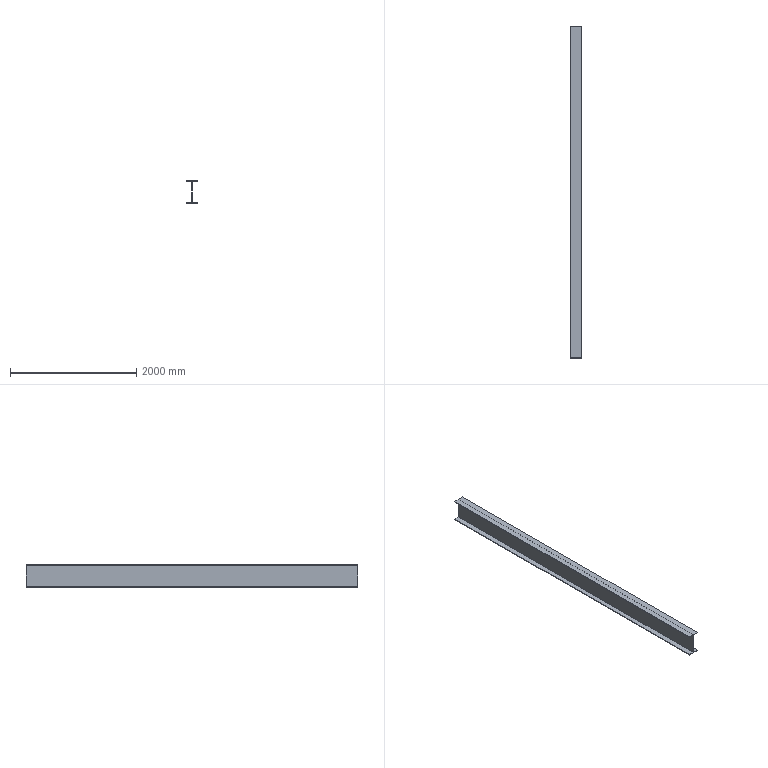Component | NX | ZHIJIA11 | 1 solid | 14 faces | box 175 x 5250 x 350 mm | volume 35700000 mm3 | plane 14
STEP:
#1=CARTESIAN_POINT('',(0.,0.,0.));
#2=DIRECTION('',(0.,0.,1.));
#3=DIRECTION('',(1.,0.,0.));
#4=AXIS2_PLACEMENT_3D('',#1,#2,#3);
#5=CARTESIAN_POINT('',(2412.5,2625.,3538.094));
#6=VERTEX_POINT('',#5);
#7=CARTESIAN_POINT('',(2412.5,2625.,3528.094));
#8=VERTEX_POINT('',#7);
#9=CARTESIAN_POINT('',(2412.5,2625.,3538.094));
#10=DIRECTION('',(-0.,0.,-1.));
#11=VECTOR('',#10,1.);
#12=LINE('',#9,#11);
#13=CARTESIAN_POINT('',(2412.5,-2625.,3538.094));
#14=DIRECTION('',(1.,0.,-0.));
#15=DIRECTION('',(0.,0.,1.));
#16=AXIS2_PLACEMENT_3D('',#13,#14,#15);
#17=PLANE('',#16);
#18=CARTESIAN_POINT('',(0.,-5250.));
#19=DIRECTION('',(-1.,0.));
#20=VECTOR('',#19,1.);
#21=LINE('',#18,#20);
#22=(GEOMETRIC_REPRESENTATION_CONTEXT(2)PARAMETRIC_REPRESENTATION_CONTEXT()REPRESENTATION_CONTEXT('',''));
#23=DEFINITIONAL_REPRESENTATION('',(#21),#22);
#24=PCURVE('',#17,#23);
#25=CARTESIAN_POINT('',(2412.5,2625.,3528.094));
#26=DIRECTION('',(0.,-1.,0.));
#27=DIRECTION('',(1.,0.,0.));
#28=AXIS2_PLACEMENT_3D('',#25,#26,#27);
#29=PLANE('',#28);
#30=CARTESIAN_POINT('',(0.,10.));
#31=DIRECTION('',(-0.,-1.));
#32=VECTOR('',#31,1.);
#33=LINE('',#30,#32);
#34=(GEOMETRIC_REPRESENTATION_CONTEXT(2)PARAMETRIC_REPRESENTATION_CONTEXT()REPRESENTATION_CONTEXT('',''));
#35=DEFINITIONAL_REPRESENTATION('',(#33),#34);
#36=PCURVE('',#29,#35);
#37=SURFACE_CURVE('',#12,(#24,#36),.PCURVE_S1.);
#38=EDGE_CURVE('',#6,#8,#37,.T.);
#39=ORIENTED_EDGE('',*,*,#38,.T.);
#40=CARTESIAN_POINT('',(2412.5,-2625.,3528.094));
#41=VERTEX_POINT('',#40);
#42=CARTESIAN_POINT('',(2412.5,-2625.,3528.094));
#43=DIRECTION('',(0.,1.,0.));
#44=VECTOR('',#43,1.);
#45=LINE('',#42,#44);
#46=CARTESIAN_POINT('',(-10.,0.));
#47=DIRECTION('',(0.,-1.));
#48=VECTOR('',#47,1.);
#49=LINE('',#46,#48);
#50=(GEOMETRIC_REPRESENTATION_CONTEXT(2)PARAMETRIC_REPRESENTATION_CONTEXT()REPRESENTATION_CONTEXT('',''));
#51=DEFINITIONAL_REPRESENTATION('',(#49),#50);
#52=PCURVE('',#17,#51);
#53=CARTESIAN_POINT('',(2412.5,-2625.,3528.094));
#54=DIRECTION('',(0.,0.,1.));
#55=DIRECTION('',(0.,-1.,0.));
#56=AXIS2_PLACEMENT_3D('',#53,#54,#55);
#57=PLANE('',#56);
#58=CARTESIAN_POINT('',(0.,0.));
#59=DIRECTION('',(-1.,0.));
#60=VECTOR('',#59,1.);
#61=LINE('',#58,#60);
#62=(GEOMETRIC_REPRESENTATION_CONTEXT(2)PARAMETRIC_REPRESENTATION_CONTEXT()REPRESENTATION_CONTEXT('',''));
#63=DEFINITIONAL_REPRESENTATION('',(#61),#62);
#64=PCURVE('',#57,#63);
#65=SURFACE_CURVE('',#45,(#52,#64),.PCURVE_S1.);
#66=EDGE_CURVE('',#41,#8,#65,.T.);
#67=ORIENTED_EDGE('',*,*,#66,.F.);
#68=CARTESIAN_POINT('',(2412.5,-2625.,3538.094));
#69=VERTEX_POINT('',#68);
#70=CARTESIAN_POINT('',(2412.5,-2625.,3538.094));
#71=DIRECTION('',(-0.,0.,-1.));
#72=VECTOR('',#71,1.);
#73=LINE('',#70,#72);
#74=CARTESIAN_POINT('',(0.,0.));
#75=DIRECTION('',(-1.,0.));
#76=VECTOR('',#75,1.);
#77=LINE('',#74,#76);
#78=(GEOMETRIC_REPRESENTATION_CONTEXT(2)PARAMETRIC_REPRESENTATION_CONTEXT()REPRESENTATION_CONTEXT('',''));
#79=DEFINITIONAL_REPRESENTATION('',(#77),#78);
#80=PCURVE('',#17,#79);
#81=CARTESIAN_POINT('',(2412.5,-2625.,3528.094));
#82=DIRECTION('',(0.,-1.,0.));
#83=DIRECTION('',(1.,0.,0.));
#84=AXIS2_PLACEMENT_3D('',#81,#82,#83);
#85=PLANE('',#84);
#86=CARTESIAN_POINT('',(0.,10.));
#87=DIRECTION('',(-0.,-1.));
#88=VECTOR('',#87,1.);
#89=LINE('',#86,#88);
#90=(GEOMETRIC_REPRESENTATION_CONTEXT(2)PARAMETRIC_REPRESENTATION_CONTEXT()REPRESENTATION_CONTEXT('',''));
#91=DEFINITIONAL_REPRESENTATION('',(#89),#90);
#92=PCURVE('',#85,#91);
#93=SURFACE_CURVE('',#73,(#80,#92),.PCURVE_S1.);
#94=EDGE_CURVE('',#69,#41,#93,.T.);
#95=ORIENTED_EDGE('',*,*,#94,.F.);
#96=CARTESIAN_POINT('',(2412.5,-2625.,3538.094));
#97=DIRECTION('',(0.,1.,0.));
#98=VECTOR('',#97,1.);
#99=LINE('',#96,#98);
#100=CARTESIAN_POINT('',(0.,0.));
#101=DIRECTION('',(0.,-1.));
#102=VECTOR('',#101,1.);
#103=LINE('',#100,#102);
#104=(GEOMETRIC_REPRESENTATION_CONTEXT(2)PARAMETRIC_REPRESENTATION_CONTEXT()REPRESENTATION_CONTEXT('',''));
#105=DEFINITIONAL_REPRESENTATION('',(#103),#104);
#106=PCURVE('',#17,#105);
#107=CARTESIAN_POINT('',(2495.,-2625.,3538.094));
#108=DIRECTION('',(0.,0.,-1.));
#109=DIRECTION('',(0.,1.,0.));
#110=AXIS2_PLACEMENT_3D('',#107,#108,#109);
#111=PLANE('',#110);
#112=CARTESIAN_POINT('',(0.,-82.5));
#113=DIRECTION('',(1.,0.));
#114=VECTOR('',#113,1.);
#115=LINE('',#112,#114);
#116=(GEOMETRIC_REPRESENTATION_CONTEXT(2)PARAMETRIC_REPRESENTATION_CONTEXT()REPRESENTATION_CONTEXT('',''));
#117=DEFINITIONAL_REPRESENTATION('',(#115),#116);
#118=PCURVE('',#111,#117);
#119=SURFACE_CURVE('',#99,(#106,#118),.PCURVE_S1.);
#120=EDGE_CURVE('',#69,#6,#119,.T.);
#121=ORIENTED_EDGE('',*,*,#120,.T.);
#122=EDGE_LOOP('',(#39,#67,#95,#121));
#123=FACE_BOUND('',#122,.T.);
#124=ADVANCED_FACE('',(#123),#17,.F.);
#125=CARTESIAN_POINT('',(2587.5,2625.,3528.094));
#126=VERTEX_POINT('',#125);
#127=CARTESIAN_POINT('',(2412.5,2625.,3528.094));
#128=DIRECTION('',(1.,0.,0.));
#129=VECTOR('',#128,1.);
#130=LINE('',#127,#129);
#131=CARTESIAN_POINT('',(-5250.,0.));
#132=DIRECTION('',(0.,1.));
#133=VECTOR('',#132,1.);
#134=LINE('',#131,#133);
#135=(GEOMETRIC_REPRESENTATION_CONTEXT(2)PARAMETRIC_REPRESENTATION_CONTEXT()REPRESENTATION_CONTEXT('',''));
#136=DEFINITIONAL_REPRESENTATION('',(#134),#135);
#137=PCURVE('',#57,#136);
#138=CARTESIAN_POINT('',(0.,0.));
#139=DIRECTION('',(1.,0.));
#140=VECTOR('',#139,1.);
#141=LINE('',#138,#140);
#142=(GEOMETRIC_REPRESENTATION_CONTEXT(2)PARAMETRIC_REPRESENTATION_CONTEXT()REPRESENTATION_CONTEXT('',''));
#143=DEFINITIONAL_REPRESENTATION('',(#141),#142);
#144=PCURVE('',#29,#143);
#145=SURFACE_CURVE('',#130,(#137,#144),.PCURVE_S1.);
#146=EDGE_CURVE('',#8,#126,#145,.T.);
#147=ORIENTED_EDGE('',*,*,#146,.T.);
#148=CARTESIAN_POINT('',(2587.5,-2625.,3528.094));
#149=VERTEX_POINT('',#148);
#150=CARTESIAN_POINT('',(2587.5,-2625.,3528.094));
#151=DIRECTION('',(0.,1.,0.));
#152=VECTOR('',#151,1.);
#153=LINE('',#150,#152);
#154=CARTESIAN_POINT('',(0.,175.));
#155=DIRECTION('',(-1.,0.));
#156=VECTOR('',#155,1.);
#157=LINE('',#154,#156);
#158=(GEOMETRIC_REPRESENTATION_CONTEXT(2)PARAMETRIC_REPRESENTATION_CONTEXT()REPRESENTATION_CONTEXT('',''));
#159=DEFINITIONAL_REPRESENTATION('',(#157),#158);
#160=PCURVE('',#57,#159);
#161=CARTESIAN_POINT('',(2587.5,-2625.,3528.094));
#162=DIRECTION('',(-1.,0.,0.));
#163=DIRECTION('',(-0.,0.,-1.));
#164=AXIS2_PLACEMENT_3D('',#161,#162,#163);
#165=PLANE('',#164);
#166=CARTESIAN_POINT('',(0.,0.));
#167=DIRECTION('',(0.,-1.));
#168=VECTOR('',#167,1.);
#169=LINE('',#166,#168);
#170=(GEOMETRIC_REPRESENTATION_CONTEXT(2)PARAMETRIC_REPRESENTATION_CONTEXT()REPRESENTATION_CONTEXT('',''));
#171=DEFINITIONAL_REPRESENTATION('',(#169),#170);
#172=PCURVE('',#165,#171);
#173=SURFACE_CURVE('',#153,(#160,#172),.PCURVE_S1.);
#174=EDGE_CURVE('',#149,#126,#173,.T.);
#175=ORIENTED_EDGE('',*,*,#174,.F.);
#176=CARTESIAN_POINT('',(2412.5,-2625.,3528.094));
#177=DIRECTION('',(1.,0.,0.));
#178=VECTOR('',#177,1.);
#179=LINE('',#176,#178);
#180=CARTESIAN_POINT('',(0.,0.));
#181=DIRECTION('',(0.,1.));
#182=VECTOR('',#181,1.);
#183=LINE('',#180,#182);
#184=(GEOMETRIC_REPRESENTATION_CONTEXT(2)PARAMETRIC_REPRESENTATION_CONTEXT()REPRESENTATION_CONTEXT('',''));
#185=DEFINITIONAL_REPRESENTATION('',(#183),#184);
#186=PCURVE('',#57,#185);
#187=CARTESIAN_POINT('',(0.,0.));
#188=DIRECTION('',(1.,0.));
#189=VECTOR('',#188,1.);
#190=LINE('',#187,#189);
#191=(GEOMETRIC_REPRESENTATION_CONTEXT(2)PARAMETRIC_REPRESENTATION_CONTEXT()REPRESENTATION_CONTEXT('',''));
#192=DEFINITIONAL_REPRESENTATION('',(#190),#191);
#193=PCURVE('',#85,#192);
#194=SURFACE_CURVE('',#179,(#186,#193),.PCURVE_S1.);
#195=EDGE_CURVE('',#41,#149,#194,.T.);
#196=ORIENTED_EDGE('',*,*,#195,.F.);
#197=ORIENTED_EDGE('',*,*,#66,.T.);
#198=EDGE_LOOP('',(#147,#175,#196,#197));
#199=FACE_BOUND('',#198,.T.);
#200=ADVANCED_FACE('',(#199),#57,.F.);
#201=CARTESIAN_POINT('',(2587.5,2625.,3538.094));
#202=VERTEX_POINT('',#201);
#203=CARTESIAN_POINT('',(2587.5,2625.,3528.094));
#204=DIRECTION('',(0.,0.,1.));
#205=VECTOR('',#204,1.);
#206=LINE('',#203,#205);
#207=CARTESIAN_POINT('',(0.,-5250.));
#208=DIRECTION('',(-1.,0.));
#209=VECTOR('',#208,1.);
#210=LINE('',#207,#209);
#211=(GEOMETRIC_REPRESENTATION_CONTEXT(2)PARAMETRIC_REPRESENTATION_CONTEXT()REPRESENTATION_CONTEXT('',''));
#212=DEFINITIONAL_REPRESENTATION('',(#210),#211);
#213=PCURVE('',#165,#212);
#214=CARTESIAN_POINT('',(175.,0.));
#215=DIRECTION('',(0.,1.));
#216=VECTOR('',#215,1.);
#217=LINE('',#214,#216);
#218=(GEOMETRIC_REPRESENTATION_CONTEXT(2)PARAMETRIC_REPRESENTATION_CONTEXT()REPRESENTATION_CONTEXT('',''));
#219=DEFINITIONAL_REPRESENTATION('',(#217),#218);
#220=PCURVE('',#29,#219);
#221=SURFACE_CURVE('',#206,(#213,#220),.PCURVE_S1.);
#222=EDGE_CURVE('',#126,#202,#221,.T.);
#223=ORIENTED_EDGE('',*,*,#222,.T.);
#224=CARTESIAN_POINT('',(2587.5,-2625.,3538.094));
#225=VERTEX_POINT('',#224);
#226=CARTESIAN_POINT('',(2587.5,-2625.,3538.094));
#227=DIRECTION('',(0.,1.,0.));
#228=VECTOR('',#227,1.);
#229=LINE('',#226,#228);
#230=CARTESIAN_POINT('',(-10.,0.));
#231=DIRECTION('',(0.,-1.));
#232=VECTOR('',#231,1.);
#233=LINE('',#230,#232);
#234=(GEOMETRIC_REPRESENTATION_CONTEXT(2)PARAMETRIC_REPRESENTATION_CONTEXT()REPRESENTATION_CONTEXT('',''));
#235=DEFINITIONAL_REPRESENTATION('',(#233),#234);
#236=PCURVE('',#165,#235);
#237=CARTESIAN_POINT('',(2587.5,-2625.,3538.094));
#238=DIRECTION('',(0.,0.,-1.));
#239=DIRECTION('',(0.,1.,0.));
#240=AXIS2_PLACEMENT_3D('',#237,#238,#239);
#241=PLANE('',#240);
#242=CARTESIAN_POINT('',(0.,0.));
#243=DIRECTION('',(1.,0.));
#244=VECTOR('',#243,1.);
#245=LINE('',#242,#244);
#246=(GEOMETRIC_REPRESENTATION_CONTEXT(2)PARAMETRIC_REPRESENTATION_CONTEXT()REPRESENTATION_CONTEXT('',''));
#247=DEFINITIONAL_REPRESENTATION('',(#245),#246);
#248=PCURVE('',#241,#247);
#249=SURFACE_CURVE('',#229,(#236,#248),.PCURVE_S1.);
#250=EDGE_CURVE('',#225,#202,#249,.T.);
#251=ORIENTED_EDGE('',*,*,#250,.F.);
#252=CARTESIAN_POINT('',(2587.5,-2625.,3528.094));
#253=DIRECTION('',(0.,0.,1.));
#254=VECTOR('',#253,1.);
#255=LINE('',#252,#254);
#256=CARTESIAN_POINT('',(0.,0.));
#257=DIRECTION('',(-1.,0.));
#258=VECTOR('',#257,1.);
#259=LINE('',#256,#258);
#260=(GEOMETRIC_REPRESENTATION_CONTEXT(2)PARAMETRIC_REPRESENTATION_CONTEXT()REPRESENTATION_CONTEXT('',''));
#261=DEFINITIONAL_REPRESENTATION('',(#259),#260);
#262=PCURVE('',#165,#261);
#263=CARTESIAN_POINT('',(175.,0.));
#264=DIRECTION('',(0.,1.));
#265=VECTOR('',#264,1.);
#266=LINE('',#263,#265);
#267=(GEOMETRIC_REPRESENTATION_CONTEXT(2)PARAMETRIC_REPRESENTATION_CONTEXT()REPRESENTATION_CONTEXT('',''));
#268=DEFINITIONAL_REPRESENTATION('',(#266),#267);
#269=PCURVE('',#85,#268);
#270=SURFACE_CURVE('',#255,(#262,#269),.PCURVE_S1.);
#271=EDGE_CURVE('',#149,#225,#270,.T.);
#272=ORIENTED_EDGE('',*,*,#271,.F.);
#273=ORIENTED_EDGE('',*,*,#174,.T.);
#274=EDGE_LOOP('',(#223,#251,#272,#273));
#275=FACE_BOUND('',#274,.T.);
#276=ADVANCED_FACE('',(#275),#165,.F.);
#277=CARTESIAN_POINT('',(2505.,2625.,3538.094));
#278=VERTEX_POINT('',#277);
#279=CARTESIAN_POINT('',(2587.5,2625.,3538.094));
#280=DIRECTION('',(-1.,0.,0.));
#281=VECTOR('',#280,1.);
#282=LINE('',#279,#281);
#283=CARTESIAN_POINT('',(5250.,0.));
#284=DIRECTION('',(0.,-1.));
#285=VECTOR('',#284,1.);
#286=LINE('',#283,#285);
#287=(GEOMETRIC_REPRESENTATION_CONTEXT(2)PARAMETRIC_REPRESENTATION_CONTEXT()REPRESENTATION_CONTEXT('',''));
#288=DEFINITIONAL_REPRESENTATION('',(#286),#287);
#289=PCURVE('',#241,#288);
#290=CARTESIAN_POINT('',(175.,10.));
#291=DIRECTION('',(-1.,0.));
#292=VECTOR('',#291,1.);
#293=LINE('',#290,#292);
#294=(GEOMETRIC_REPRESENTATION_CONTEXT(2)PARAMETRIC_REPRESENTATION_CONTEXT()REPRESENTATION_CONTEXT('',''));
#295=DEFINITIONAL_REPRESENTATION('',(#293),#294);
#296=PCURVE('',#29,#295);
#297=SURFACE_CURVE('',#282,(#289,#296),.PCURVE_S1.);
#298=EDGE_CURVE('',#202,#278,#297,.T.);
#299=ORIENTED_EDGE('',*,*,#298,.T.);
#300=CARTESIAN_POINT('',(2505.,-2625.,3538.094));
#301=VERTEX_POINT('',#300);
#302=CARTESIAN_POINT('',(2505.,-2625.,3538.094));
#303=DIRECTION('',(0.,1.,0.));
#304=VECTOR('',#303,1.);
#305=LINE('',#302,#304);
#306=CARTESIAN_POINT('',(0.,-82.5));
#307=DIRECTION('',(1.,0.));
#308=VECTOR('',#307,1.);
#309=LINE('',#306,#308);
#310=(GEOMETRIC_REPRESENTATION_CONTEXT(2)PARAMETRIC_REPRESENTATION_CONTEXT()REPRESENTATION_CONTEXT('',''));
#311=DEFINITIONAL_REPRESENTATION('',(#309),#310);
#312=PCURVE('',#241,#311);
#313=CARTESIAN_POINT('',(2505.,-2625.,3538.094));
#314=DIRECTION('',(-1.,0.,0.));
#315=DIRECTION('',(-0.,0.,-1.));
#316=AXIS2_PLACEMENT_3D('',#313,#314,#315);
#317=PLANE('',#316);
#318=CARTESIAN_POINT('',(0.,0.));
#319=DIRECTION('',(0.,-1.));
#320=VECTOR('',#319,1.);
#321=LINE('',#318,#320);
#322=(GEOMETRIC_REPRESENTATION_CONTEXT(2)PARAMETRIC_REPRESENTATION_CONTEXT()REPRESENTATION_CONTEXT('',''));
#323=DEFINITIONAL_REPRESENTATION('',(#321),#322);
#324=PCURVE('',#317,#323);
#325=SURFACE_CURVE('',#305,(#312,#324),.PCURVE_S1.);
#326=EDGE_CURVE('',#301,#278,#325,.T.);
#327=ORIENTED_EDGE('',*,*,#326,.F.);
#328=CARTESIAN_POINT('',(2587.5,-2625.,3538.094));
#329=DIRECTION('',(-1.,0.,0.));
#330=VECTOR('',#329,1.);
#331=LINE('',#328,#330);
#332=CARTESIAN_POINT('',(0.,0.));
#333=DIRECTION('',(0.,-1.));
#334=VECTOR('',#333,1.);
#335=LINE('',#332,#334);
#336=(GEOMETRIC_REPRESENTATION_CONTEXT(2)PARAMETRIC_REPRESENTATION_CONTEXT()REPRESENTATION_CONTEXT('',''));
#337=DEFINITIONAL_REPRESENTATION('',(#335),#336);
#338=PCURVE('',#241,#337);
#339=CARTESIAN_POINT('',(175.,10.));
#340=DIRECTION('',(-1.,0.));
#341=VECTOR('',#340,1.);
#342=LINE('',#339,#341);
#343=(GEOMETRIC_REPRESENTATION_CONTEXT(2)PARAMETRIC_REPRESENTATION_CONTEXT()REPRESENTATION_CONTEXT('',''));
#344=DEFINITIONAL_REPRESENTATION('',(#342),#343);
#345=PCURVE('',#85,#344);
#346=SURFACE_CURVE('',#331,(#338,#345),.PCURVE_S1.);
#347=EDGE_CURVE('',#225,#301,#346,.T.);
#348=ORIENTED_EDGE('',*,*,#347,.F.);
#349=ORIENTED_EDGE('',*,*,#250,.T.);
#350=EDGE_LOOP('',(#299,#327,#348,#349));
#351=FACE_BOUND('',#350,.T.);
#352=ADVANCED_FACE('',(#351),#241,.F.);
#353=CARTESIAN_POINT('',(2505.,2625.,3868.094));
#354=VERTEX_POINT('',#353);
#355=CARTESIAN_POINT('',(2505.,2625.,3538.094));
#356=DIRECTION('',(0.,0.,1.));
#357=VECTOR('',#356,1.);
#358=LINE('',#355,#357);
#359=CARTESIAN_POINT('',(0.,-5250.));
#360=DIRECTION('',(-1.,0.));
#361=VECTOR('',#360,1.);
#362=LINE('',#359,#361);
#363=(GEOMETRIC_REPRESENTATION_CONTEXT(2)PARAMETRIC_REPRESENTATION_CONTEXT()REPRESENTATION_CONTEXT('',''));
#364=DEFINITIONAL_REPRESENTATION('',(#362),#363);
#365=PCURVE('',#317,#364);
#366=CARTESIAN_POINT('',(92.5,10.));
#367=DIRECTION('',(0.,1.));
#368=VECTOR('',#367,1.);
#369=LINE('',#366,#368);
#370=(GEOMETRIC_REPRESENTATION_CONTEXT(2)PARAMETRIC_REPRESENTATION_CONTEXT()REPRESENTATION_CONTEXT('',''));
#371=DEFINITIONAL_REPRESENTATION('',(#369),#370);
#372=PCURVE('',#29,#371);
#373=SURFACE_CURVE('',#358,(#365,#372),.PCURVE_S1.);
#374=EDGE_CURVE('',#278,#354,#373,.T.);
#375=ORIENTED_EDGE('',*,*,#374,.T.);
#376=CARTESIAN_POINT('',(2505.,-2625.,3868.094));
#377=VERTEX_POINT('',#376);
#378=CARTESIAN_POINT('',(2505.,-2625.,3868.094));
#379=DIRECTION('',(0.,1.,0.));
#380=VECTOR('',#379,1.);
#381=LINE('',#378,#380);
#382=CARTESIAN_POINT('',(-330.,0.));
#383=DIRECTION('',(0.,-1.));
#384=VECTOR('',#383,1.);
#385=LINE('',#382,#384);
#386=(GEOMETRIC_REPRESENTATION_CONTEXT(2)PARAMETRIC_REPRESENTATION_CONTEXT()REPRESENTATION_CONTEXT('',''));
#387=DEFINITIONAL_REPRESENTATION('',(#385),#386);
#388=PCURVE('',#317,#387);
#389=CARTESIAN_POINT('',(2505.,-2625.,3868.094));
#390=DIRECTION('',(0.,0.,1.));
#391=DIRECTION('',(0.,-1.,0.));
#392=AXIS2_PLACEMENT_3D('',#389,#390,#391);
#393=PLANE('',#392);
#394=CARTESIAN_POINT('',(0.,0.));
#395=DIRECTION('',(-1.,0.));
#396=VECTOR('',#395,1.);
#397=LINE('',#394,#396);
#398=(GEOMETRIC_REPRESENTATION_CONTEXT(2)PARAMETRIC_REPRESENTATION_CONTEXT()REPRESENTATION_CONTEXT('',''));
#399=DEFINITIONAL_REPRESENTATION('',(#397),#398);
#400=PCURVE('',#393,#399);
#401=SURFACE_CURVE('',#381,(#388,#400),.PCURVE_S1.);
#402=EDGE_CURVE('',#377,#354,#401,.T.);
#403=ORIENTED_EDGE('',*,*,#402,.F.);
#404=CARTESIAN_POINT('',(2505.,-2625.,3538.094));
#405=DIRECTION('',(0.,0.,1.));
#406=VECTOR('',#405,1.);
#407=LINE('',#404,#406);
#408=CARTESIAN_POINT('',(0.,0.));
#409=DIRECTION('',(-1.,0.));
#410=VECTOR('',#409,1.);
#411=LINE('',#408,#410);
#412=(GEOMETRIC_REPRESENTATION_CONTEXT(2)PARAMETRIC_REPRESENTATION_CONTEXT()REPRESENTATION_CONTEXT('',''));
#413=DEFINITIONAL_REPRESENTATION('',(#411),#412);
#414=PCURVE('',#317,#413);
#415=CARTESIAN_POINT('',(92.5,10.));
#416=DIRECTION('',(0.,1.));
#417=VECTOR('',#416,1.);
#418=LINE('',#415,#417);
#419=(GEOMETRIC_REPRESENTATION_CONTEXT(2)PARAMETRIC_REPRESENTATION_CONTEXT()REPRESENTATION_CONTEXT('',''));
#420=DEFINITIONAL_REPRESENTATION('',(#418),#419);
#421=PCURVE('',#85,#420);
#422=SURFACE_CURVE('',#407,(#414,#421),.PCURVE_S1.);
#423=EDGE_CURVE('',#301,#377,#422,.T.);
#424=ORIENTED_EDGE('',*,*,#423,.F.);
#425=ORIENTED_EDGE('',*,*,#326,.T.);
#426=EDGE_LOOP('',(#375,#403,#424,#425));
#427=FACE_BOUND('',#426,.T.);
#428=ADVANCED_FACE('',(#427),#317,.F.);
#429=CARTESIAN_POINT('',(2587.5,2625.,3868.094));
#430=VERTEX_POINT('',#429);
#431=CARTESIAN_POINT('',(2505.,2625.,3868.094));
#432=DIRECTION('',(1.,0.,0.));
#433=VECTOR('',#432,1.);
#434=LINE('',#431,#433);
#435=CARTESIAN_POINT('',(-5250.,0.));
#436=DIRECTION('',(0.,1.));
#437=VECTOR('',#436,1.);
#438=LINE('',#435,#437);
#439=(GEOMETRIC_REPRESENTATION_CONTEXT(2)PARAMETRIC_REPRESENTATION_CONTEXT()REPRESENTATION_CONTEXT('',''));
#440=DEFINITIONAL_REPRESENTATION('',(#438),#439);
#441=PCURVE('',#393,#440);
#442=CARTESIAN_POINT('',(92.5,340.));
#443=DIRECTION('',(1.,0.));
#444=VECTOR('',#443,1.);
#445=LINE('',#442,#444);
#446=(GEOMETRIC_REPRESENTATION_CONTEXT(2)PARAMETRIC_REPRESENTATION_CONTEXT()REPRESENTATION_CONTEXT('',''));
#447=DEFINITIONAL_REPRESENTATION('',(#445),#446);
#448=PCURVE('',#29,#447);
#449=SURFACE_CURVE('',#434,(#441,#448),.PCURVE_S1.);
#450=EDGE_CURVE('',#354,#430,#449,.T.);
#451=ORIENTED_EDGE('',*,*,#450,.T.);
#452=CARTESIAN_POINT('',(2587.5,-2625.,3868.094));
#453=VERTEX_POINT('',#452);
#454=CARTESIAN_POINT('',(2587.5,-2625.,3868.094));
#455=DIRECTION('',(0.,1.,0.));
#456=VECTOR('',#455,1.);
#457=LINE('',#454,#456);
#458=CARTESIAN_POINT('',(0.,82.5));
#459=DIRECTION('',(-1.,0.));
#460=VECTOR('',#459,1.);
#461=LINE('',#458,#460);
#462=(GEOMETRIC_REPRESENTATION_CONTEXT(2)PARAMETRIC_REPRESENTATION_CONTEXT()REPRESENTATION_CONTEXT('',''));
#463=DEFINITIONAL_REPRESENTATION('',(#461),#462);
#464=PCURVE('',#393,#463);
#465=CARTESIAN_POINT('',(2587.5,-2625.,3868.094));
#466=DIRECTION('',(-1.,0.,0.));
#467=DIRECTION('',(-0.,0.,-1.));
#468=AXIS2_PLACEMENT_3D('',#465,#466,#467);
#469=PLANE('',#468);
#470=CARTESIAN_POINT('',(0.,0.));
#471=DIRECTION('',(0.,-1.));
#472=VECTOR('',#471,1.);
#473=LINE('',#470,#472);
#474=(GEOMETRIC_REPRESENTATION_CONTEXT(2)PARAMETRIC_REPRESENTATION_CONTEXT()REPRESENTATION_CONTEXT('',''));
#475=DEFINITIONAL_REPRESENTATION('',(#473),#474);
#476=PCURVE('',#469,#475);
#477=SURFACE_CURVE('',#457,(#464,#476),.PCURVE_S1.);
#478=EDGE_CURVE('',#453,#430,#477,.T.);
#479=ORIENTED_EDGE('',*,*,#478,.F.);
#480=CARTESIAN_POINT('',(2505.,-2625.,3868.094));
#481=DIRECTION('',(1.,0.,0.));
#482=VECTOR('',#481,1.);
#483=LINE('',#480,#482);
#484=CARTESIAN_POINT('',(0.,0.));
#485=DIRECTION('',(0.,1.));
#486=VECTOR('',#485,1.);
#487=LINE('',#484,#486);
#488=(GEOMETRIC_REPRESENTATION_CONTEXT(2)PARAMETRIC_REPRESENTATION_CONTEXT()REPRESENTATION_CONTEXT('',''));
#489=DEFINITIONAL_REPRESENTATION('',(#487),#488);
#490=PCURVE('',#393,#489);
#491=CARTESIAN_POINT('',(92.5,340.));
#492=DIRECTION('',(1.,0.));
#493=VECTOR('',#492,1.);
#494=LINE('',#491,#493);
#495=(GEOMETRIC_REPRESENTATION_CONTEXT(2)PARAMETRIC_REPRESENTATION_CONTEXT()REPRESENTATION_CONTEXT('',''));
#496=DEFINITIONAL_REPRESENTATION('',(#494),#495);
#497=PCURVE('',#85,#496);
#498=SURFACE_CURVE('',#483,(#490,#497),.PCURVE_S1.);
#499=EDGE_CURVE('',#377,#453,#498,.T.);
#500=ORIENTED_EDGE('',*,*,#499,.F.);
#501=ORIENTED_EDGE('',*,*,#402,.T.);
#502=EDGE_LOOP('',(#451,#479,#500,#501));
#503=FACE_BOUND('',#502,.T.);
#504=ADVANCED_FACE('',(#503),#393,.F.);
#505=CARTESIAN_POINT('',(2587.5,2625.,3878.094));
#506=VERTEX_POINT('',#505);
#507=CARTESIAN_POINT('',(2587.5,2625.,3868.094));
#508=DIRECTION('',(0.,0.,1.));
#509=VECTOR('',#508,1.);
#510=LINE('',#507,#509);
#511=CARTESIAN_POINT('',(0.,-5250.));
#512=DIRECTION('',(-1.,0.));
#513=VECTOR('',#512,1.);
#514=LINE('',#511,#513);
#515=(GEOMETRIC_REPRESENTATION_CONTEXT(2)PARAMETRIC_REPRESENTATION_CONTEXT()REPRESENTATION_CONTEXT('',''));
#516=DEFINITIONAL_REPRESENTATION('',(#514),#515);
#517=PCURVE('',#469,#516);
#518=CARTESIAN_POINT('',(175.,340.));
#519=DIRECTION('',(0.,1.));
#520=VECTOR('',#519,1.);
#521=LINE('',#518,#520);
#522=(GEOMETRIC_REPRESENTATION_CONTEXT(2)PARAMETRIC_REPRESENTATION_CONTEXT()REPRESENTATION_CONTEXT('',''));
#523=DEFINITIONAL_REPRESENTATION('',(#521),#522);
#524=PCURVE('',#29,#523);
#525=SURFACE_CURVE('',#510,(#517,#524),.PCURVE_S1.);
#526=EDGE_CURVE('',#430,#506,#525,.T.);
#527=ORIENTED_EDGE('',*,*,#526,.T.);
#528=CARTESIAN_POINT('',(2587.5,-2625.,3878.094));
#529=VERTEX_POINT('',#528);
#530=CARTESIAN_POINT('',(2587.5,-2625.,3878.094));
#531=DIRECTION('',(0.,1.,0.));
#532=VECTOR('',#531,1.);
#533=LINE('',#530,#532);
#534=CARTESIAN_POINT('',(-10.,0.));
#535=DIRECTION('',(0.,-1.));
#536=VECTOR('',#535,1.);
#537=LINE('',#534,#536);
#538=(GEOMETRIC_REPRESENTATION_CONTEXT(2)PARAMETRIC_REPRESENTATION_CONTEXT()REPRESENTATION_CONTEXT('',''));
#539=DEFINITIONAL_REPRESENTATION('',(#537),#538);
#540=PCURVE('',#469,#539);
#541=CARTESIAN_POINT('',(2587.5,-2625.,3878.094));
#542=DIRECTION('',(0.,0.,-1.));
#543=DIRECTION('',(0.,1.,0.));
#544=AXIS2_PLACEMENT_3D('',#541,#542,#543);
#545=PLANE('',#544);
#546=CARTESIAN_POINT('',(0.,0.));
#547=DIRECTION('',(1.,0.));
#548=VECTOR('',#547,1.);
#549=LINE('',#546,#548);
#550=(GEOMETRIC_REPRESENTATION_CONTEXT(2)PARAMETRIC_REPRESENTATION_CONTEXT()REPRESENTATION_CONTEXT('',''));
#551=DEFINITIONAL_REPRESENTATION('',(#549),#550);
#552=PCURVE('',#545,#551);
#553=SURFACE_CURVE('',#533,(#540,#552),.PCURVE_S1.);
#554=EDGE_CURVE('',#529,#506,#553,.T.);
#555=ORIENTED_EDGE('',*,*,#554,.F.);
#556=CARTESIAN_POINT('',(2587.5,-2625.,3868.094));
#557=DIRECTION('',(0.,0.,1.));
#558=VECTOR('',#557,1.);
#559=LINE('',#556,#558);
#560=CARTESIAN_POINT('',(0.,0.));
#561=DIRECTION('',(-1.,0.));
#562=VECTOR('',#561,1.);
#563=LINE('',#560,#562);
#564=(GEOMETRIC_REPRESENTATION_CONTEXT(2)PARAMETRIC_REPRESENTATION_CONTEXT()REPRESENTATION_CONTEXT('',''));
#565=DEFINITIONAL_REPRESENTATION('',(#563),#564);
#566=PCURVE('',#469,#565);
#567=CARTESIAN_POINT('',(175.,340.));
#568=DIRECTION('',(0.,1.));
#569=VECTOR('',#568,1.);
#570=LINE('',#567,#569);
#571=(GEOMETRIC_REPRESENTATION_CONTEXT(2)PARAMETRIC_REPRESENTATION_CONTEXT()REPRESENTATION_CONTEXT('',''));
#572=DEFINITIONAL_REPRESENTATION('',(#570),#571);
#573=PCURVE('',#85,#572);
#574=SURFACE_CURVE('',#559,(#566,#573),.PCURVE_S1.);
#575=EDGE_CURVE('',#453,#529,#574,.T.);
#576=ORIENTED_EDGE('',*,*,#575,.F.);
#577=ORIENTED_EDGE('',*,*,#478,.T.);
#578=EDGE_LOOP('',(#527,#555,#576,#577));
#579=FACE_BOUND('',#578,.T.);
#580=ADVANCED_FACE('',(#579),#469,.F.);
#581=CARTESIAN_POINT('',(2412.5,2625.,3878.094));
#582=VERTEX_POINT('',#581);
#583=CARTESIAN_POINT('',(2587.5,2625.,3878.094));
#584=DIRECTION('',(-1.,0.,0.));
#585=VECTOR('',#584,1.);
#586=LINE('',#583,#585);
#587=CARTESIAN_POINT('',(5250.,0.));
#588=DIRECTION('',(0.,-1.));
#589=VECTOR('',#588,1.);
#590=LINE('',#587,#589);
#591=(GEOMETRIC_REPRESENTATION_CONTEXT(2)PARAMETRIC_REPRESENTATION_CONTEXT()REPRESENTATION_CONTEXT('',''));
#592=DEFINITIONAL_REPRESENTATION('',(#590),#591);
#593=PCURVE('',#545,#592);
#594=CARTESIAN_POINT('',(175.,350.));
#595=DIRECTION('',(-1.,0.));
#596=VECTOR('',#595,1.);
#597=LINE('',#594,#596);
#598=(GEOMETRIC_REPRESENTATION_CONTEXT(2)PARAMETRIC_REPRESENTATION_CONTEXT()REPRESENTATION_CONTEXT('',''));
#599=DEFINITIONAL_REPRESENTATION('',(#597),#598);
#600=PCURVE('',#29,#599);
#601=SURFACE_CURVE('',#586,(#593,#600),.PCURVE_S1.);
#602=EDGE_CURVE('',#506,#582,#601,.T.);
#603=ORIENTED_EDGE('',*,*,#602,.T.);
#604=CARTESIAN_POINT('',(2412.5,-2625.,3878.094));
#605=VERTEX_POINT('',#604);
#606=CARTESIAN_POINT('',(2412.5,-2625.,3878.094));
#607=DIRECTION('',(0.,1.,0.));
#608=VECTOR('',#607,1.);
#609=LINE('',#606,#608);
#610=CARTESIAN_POINT('',(0.,-175.));
#611=DIRECTION('',(1.,0.));
#612=VECTOR('',#611,1.);
#613=LINE('',#610,#612);
#614=(GEOMETRIC_REPRESENTATION_CONTEXT(2)PARAMETRIC_REPRESENTATION_CONTEXT()REPRESENTATION_CONTEXT('',''));
#615=DEFINITIONAL_REPRESENTATION('',(#613),#614);
#616=PCURVE('',#545,#615);
#617=CARTESIAN_POINT('',(2412.5,-2625.,3878.094));
#618=DIRECTION('',(1.,0.,-0.));
#619=DIRECTION('',(0.,0.,1.));
#620=AXIS2_PLACEMENT_3D('',#617,#618,#619);
#621=PLANE('',#620);
#622=CARTESIAN_POINT('',(0.,0.));
#623=DIRECTION('',(0.,-1.));
#624=VECTOR('',#623,1.);
#625=LINE('',#622,#624);
#626=(GEOMETRIC_REPRESENTATION_CONTEXT(2)PARAMETRIC_REPRESENTATION_CONTEXT()REPRESENTATION_CONTEXT('',''));
#627=DEFINITIONAL_REPRESENTATION('',(#625),#626);
#628=PCURVE('',#621,#627);
#629=SURFACE_CURVE('',#609,(#616,#628),.PCURVE_S1.);
#630=EDGE_CURVE('',#605,#582,#629,.T.);
#631=ORIENTED_EDGE('',*,*,#630,.F.);
#632=CARTESIAN_POINT('',(2587.5,-2625.,3878.094));
#633=DIRECTION('',(-1.,0.,0.));
#634=VECTOR('',#633,1.);
#635=LINE('',#632,#634);
#636=CARTESIAN_POINT('',(0.,0.));
#637=DIRECTION('',(0.,-1.));
#638=VECTOR('',#637,1.);
#639=LINE('',#636,#638);
#640=(GEOMETRIC_REPRESENTATION_CONTEXT(2)PARAMETRIC_REPRESENTATION_CONTEXT()REPRESENTATION_CONTEXT('',''));
#641=DEFINITIONAL_REPRESENTATION('',(#639),#640);
#642=PCURVE('',#545,#641);
#643=CARTESIAN_POINT('',(175.,350.));
#644=DIRECTION('',(-1.,0.));
#645=VECTOR('',#644,1.);
#646=LINE('',#643,#645);
#647=(GEOMETRIC_REPRESENTATION_CONTEXT(2)PARAMETRIC_REPRESENTATION_CONTEXT()REPRESENTATION_CONTEXT('',''));
#648=DEFINITIONAL_REPRESENTATION('',(#646),#647);
#649=PCURVE('',#85,#648);
#650=SURFACE_CURVE('',#635,(#642,#649),.PCURVE_S1.);
#651=EDGE_CURVE('',#529,#605,#650,.T.);
#652=ORIENTED_EDGE('',*,*,#651,.F.);
#653=ORIENTED_EDGE('',*,*,#554,.T.);
#654=EDGE_LOOP('',(#603,#631,#652,#653));
#655=FACE_BOUND('',#654,.T.);
#656=ADVANCED_FACE('',(#655),#545,.F.);
#657=CARTESIAN_POINT('',(2412.5,2625.,3868.094));
#658=VERTEX_POINT('',#657);
#659=CARTESIAN_POINT('',(2412.5,2625.,3878.094));
#660=DIRECTION('',(-0.,0.,-1.));
#661=VECTOR('',#660,1.);
#662=LINE('',#659,#661);
#663=CARTESIAN_POINT('',(0.,-5250.));
#664=DIRECTION('',(-1.,0.));
#665=VECTOR('',#664,1.);
#666=LINE('',#663,#665);
#667=(GEOMETRIC_REPRESENTATION_CONTEXT(2)PARAMETRIC_REPRESENTATION_CONTEXT()REPRESENTATION_CONTEXT('',''));
#668=DEFINITIONAL_REPRESENTATION('',(#666),#667);
#669=PCURVE('',#621,#668);
#670=CARTESIAN_POINT('',(0.,350.));
#671=DIRECTION('',(-0.,-1.));
#672=VECTOR('',#671,1.);
#673=LINE('',#670,#672);
#674=(GEOMETRIC_REPRESENTATION_CONTEXT(2)PARAMETRIC_REPRESENTATION_CONTEXT()REPRESENTATION_CONTEXT('',''));
#675=DEFINITIONAL_REPRESENTATION('',(#673),#674);
#676=PCURVE('',#29,#675);
#677=SURFACE_CURVE('',#662,(#669,#676),.PCURVE_S1.);
#678=EDGE_CURVE('',#582,#658,#677,.T.);
#679=ORIENTED_EDGE('',*,*,#678,.T.);
#680=CARTESIAN_POINT('',(2412.5,-2625.,3868.094));
#681=VERTEX_POINT('',#680);
#682=CARTESIAN_POINT('',(2412.5,-2625.,3868.094));
#683=DIRECTION('',(0.,1.,0.));
#684=VECTOR('',#683,1.);
#685=LINE('',#682,#684);
#686=CARTESIAN_POINT('',(-10.,0.));
#687=DIRECTION('',(0.,-1.));
#688=VECTOR('',#687,1.);
#689=LINE('',#686,#688);
#690=(GEOMETRIC_REPRESENTATION_CONTEXT(2)PARAMETRIC_REPRESENTATION_CONTEXT()REPRESENTATION_CONTEXT('',''));
#691=DEFINITIONAL_REPRESENTATION('',(#689),#690);
#692=PCURVE('',#621,#691);
#693=CARTESIAN_POINT('',(2412.5,-2625.,3868.094));
#694=DIRECTION('',(0.,0.,1.));
#695=DIRECTION('',(0.,-1.,0.));
#696=AXIS2_PLACEMENT_3D('',#693,#694,#695);
#697=PLANE('',#696);
#698=CARTESIAN_POINT('',(0.,0.));
#699=DIRECTION('',(-1.,0.));
#700=VECTOR('',#699,1.);
#701=LINE('',#698,#700);
#702=(GEOMETRIC_REPRESENTATION_CONTEXT(2)PARAMETRIC_REPRESENTATION_CONTEXT()REPRESENTATION_CONTEXT('',''));
#703=DEFINITIONAL_REPRESENTATION('',(#701),#702);
#704=PCURVE('',#697,#703);
#705=SURFACE_CURVE('',#685,(#692,#704),.PCURVE_S1.);
#706=EDGE_CURVE('',#681,#658,#705,.T.);
#707=ORIENTED_EDGE('',*,*,#706,.F.);
#708=CARTESIAN_POINT('',(2412.5,-2625.,3878.094));
#709=DIRECTION('',(-0.,0.,-1.));
#710=VECTOR('',#709,1.);
#711=LINE('',#708,#710);
#712=CARTESIAN_POINT('',(0.,0.));
#713=DIRECTION('',(-1.,0.));
#714=VECTOR('',#713,1.);
#715=LINE('',#712,#714);
#716=(GEOMETRIC_REPRESENTATION_CONTEXT(2)PARAMETRIC_REPRESENTATION_CONTEXT()REPRESENTATION_CONTEXT('',''));
#717=DEFINITIONAL_REPRESENTATION('',(#715),#716);
#718=PCURVE('',#621,#717);
#719=CARTESIAN_POINT('',(0.,350.));
#720=DIRECTION('',(-0.,-1.));
#721=VECTOR('',#720,1.);
#722=LINE('',#719,#721);
#723=(GEOMETRIC_REPRESENTATION_CONTEXT(2)PARAMETRIC_REPRESENTATION_CONTEXT()REPRESENTATION_CONTEXT('',''));
#724=DEFINITIONAL_REPRESENTATION('',(#722),#723);
#725=PCURVE('',#85,#724);
#726=SURFACE_CURVE('',#711,(#718,#725),.PCURVE_S1.);
#727=EDGE_CURVE('',#605,#681,#726,.T.);
#728=ORIENTED_EDGE('',*,*,#727,.F.);
#729=ORIENTED_EDGE('',*,*,#630,.T.);
#730=EDGE_LOOP('',(#679,#707,#728,#729));
#731=FACE_BOUND('',#730,.T.);
#732=ADVANCED_FACE('',(#731),#621,.F.);
#733=CARTESIAN_POINT('',(2495.,2625.,3868.094));
#734=VERTEX_POINT('',#733);
#735=CARTESIAN_POINT('',(2412.5,2625.,3868.094));
#736=DIRECTION('',(1.,0.,0.));
#737=VECTOR('',#736,1.);
#738=LINE('',#735,#737);
#739=CARTESIAN_POINT('',(-5250.,0.));
#740=DIRECTION('',(0.,1.));
#741=VECTOR('',#740,1.);
#742=LINE('',#739,#741);
#743=(GEOMETRIC_REPRESENTATION_CONTEXT(2)PARAMETRIC_REPRESENTATION_CONTEXT()REPRESENTATION_CONTEXT('',''));
#744=DEFINITIONAL_REPRESENTATION('',(#742),#743);
#745=PCURVE('',#697,#744);
#746=CARTESIAN_POINT('',(0.,340.));
#747=DIRECTION('',(1.,0.));
#748=VECTOR('',#747,1.);
#749=LINE('',#746,#748);
#750=(GEOMETRIC_REPRESENTATION_CONTEXT(2)PARAMETRIC_REPRESENTATION_CONTEXT()REPRESENTATION_CONTEXT('',''));
#751=DEFINITIONAL_REPRESENTATION('',(#749),#750);
#752=PCURVE('',#29,#751);
#753=SURFACE_CURVE('',#738,(#745,#752),.PCURVE_S1.);
#754=EDGE_CURVE('',#658,#734,#753,.T.);
#755=ORIENTED_EDGE('',*,*,#754,.T.);
#756=CARTESIAN_POINT('',(2495.,-2625.,3868.094));
#757=VERTEX_POINT('',#756);
#758=CARTESIAN_POINT('',(2495.,-2625.,3868.094));
#759=DIRECTION('',(0.,1.,0.));
#760=VECTOR('',#759,1.);
#761=LINE('',#758,#760);
#762=CARTESIAN_POINT('',(0.,82.5));
#763=DIRECTION('',(-1.,0.));
#764=VECTOR('',#763,1.);
#765=LINE('',#762,#764);
#766=(GEOMETRIC_REPRESENTATION_CONTEXT(2)PARAMETRIC_REPRESENTATION_CONTEXT()REPRESENTATION_CONTEXT('',''));
#767=DEFINITIONAL_REPRESENTATION('',(#765),#766);
#768=PCURVE('',#697,#767);
#769=CARTESIAN_POINT('',(2495.,-2625.,3868.094));
#770=DIRECTION('',(1.,0.,-0.));
#771=DIRECTION('',(0.,0.,1.));
#772=AXIS2_PLACEMENT_3D('',#769,#770,#771);
#773=PLANE('',#772);
#774=CARTESIAN_POINT('',(0.,0.));
#775=DIRECTION('',(0.,-1.));
#776=VECTOR('',#775,1.);
#777=LINE('',#774,#776);
#778=(GEOMETRIC_REPRESENTATION_CONTEXT(2)PARAMETRIC_REPRESENTATION_CONTEXT()REPRESENTATION_CONTEXT('',''));
#779=DEFINITIONAL_REPRESENTATION('',(#777),#778);
#780=PCURVE('',#773,#779);
#781=SURFACE_CURVE('',#761,(#768,#780),.PCURVE_S1.);
#782=EDGE_CURVE('',#757,#734,#781,.T.);
#783=ORIENTED_EDGE('',*,*,#782,.F.);
#784=CARTESIAN_POINT('',(2412.5,-2625.,3868.094));
#785=DIRECTION('',(1.,0.,0.));
#786=VECTOR('',#785,1.);
#787=LINE('',#784,#786);
#788=CARTESIAN_POINT('',(0.,0.));
#789=DIRECTION('',(0.,1.));
#790=VECTOR('',#789,1.);
#791=LINE('',#788,#790);
#792=(GEOMETRIC_REPRESENTATION_CONTEXT(2)PARAMETRIC_REPRESENTATION_CONTEXT()REPRESENTATION_CONTEXT('',''));
#793=DEFINITIONAL_REPRESENTATION('',(#791),#792);
#794=PCURVE('',#697,#793);
#795=CARTESIAN_POINT('',(0.,340.));
#796=DIRECTION('',(1.,0.));
#797=VECTOR('',#796,1.);
#798=LINE('',#795,#797);
#799=(GEOMETRIC_REPRESENTATION_CONTEXT(2)PARAMETRIC_REPRESENTATION_CONTEXT()REPRESENTATION_CONTEXT('',''));
#800=DEFINITIONAL_REPRESENTATION('',(#798),#799);
#801=PCURVE('',#85,#800);
#802=SURFACE_CURVE('',#787,(#794,#801),.PCURVE_S1.);
#803=EDGE_CURVE('',#681,#757,#802,.T.);
#804=ORIENTED_EDGE('',*,*,#803,.F.);
#805=ORIENTED_EDGE('',*,*,#706,.T.);
#806=EDGE_LOOP('',(#755,#783,#804,#805));
#807=FACE_BOUND('',#806,.T.);
#808=ADVANCED_FACE('',(#807),#697,.F.);
#809=CARTESIAN_POINT('',(2495.,2625.,3538.094));
#810=VERTEX_POINT('',#809);
#811=CARTESIAN_POINT('',(2495.,2625.,3868.094));
#812=DIRECTION('',(-0.,0.,-1.));
#813=VECTOR('',#812,1.);
#814=LINE('',#811,#813);
#815=CARTESIAN_POINT('',(0.,-5250.));
#816=DIRECTION('',(-1.,0.));
#817=VECTOR('',#816,1.);
#818=LINE('',#815,#817);
#819=(GEOMETRIC_REPRESENTATION_CONTEXT(2)PARAMETRIC_REPRESENTATION_CONTEXT()REPRESENTATION_CONTEXT('',''));
#820=DEFINITIONAL_REPRESENTATION('',(#818),#819);
#821=PCURVE('',#773,#820);
#822=CARTESIAN_POINT('',(82.5,340.));
#823=DIRECTION('',(-0.,-1.));
#824=VECTOR('',#823,1.);
#825=LINE('',#822,#824);
#826=(GEOMETRIC_REPRESENTATION_CONTEXT(2)PARAMETRIC_REPRESENTATION_CONTEXT()REPRESENTATION_CONTEXT('',''));
#827=DEFINITIONAL_REPRESENTATION('',(#825),#826);
#828=PCURVE('',#29,#827);
#829=SURFACE_CURVE('',#814,(#821,#828),.PCURVE_S1.);
#830=EDGE_CURVE('',#734,#810,#829,.T.);
#831=ORIENTED_EDGE('',*,*,#830,.T.);
#832=CARTESIAN_POINT('',(2495.,-2625.,3538.094));
#833=VERTEX_POINT('',#832);
#834=CARTESIAN_POINT('',(2495.,-2625.,3538.094));
#835=DIRECTION('',(0.,1.,0.));
#836=VECTOR('',#835,1.);
#837=LINE('',#834,#836);
#838=CARTESIAN_POINT('',(-330.,0.));
#839=DIRECTION('',(0.,-1.));
#840=VECTOR('',#839,1.);
#841=LINE('',#838,#840);
#842=(GEOMETRIC_REPRESENTATION_CONTEXT(2)PARAMETRIC_REPRESENTATION_CONTEXT()REPRESENTATION_CONTEXT('',''));
#843=DEFINITIONAL_REPRESENTATION('',(#841),#842);
#844=PCURVE('',#773,#843);
#845=CARTESIAN_POINT('',(0.,0.));
#846=DIRECTION('',(1.,0.));
#847=VECTOR('',#846,1.);
#848=LINE('',#845,#847);
#849=(GEOMETRIC_REPRESENTATION_CONTEXT(2)PARAMETRIC_REPRESENTATION_CONTEXT()REPRESENTATION_CONTEXT('',''));
#850=DEFINITIONAL_REPRESENTATION('',(#848),#849);
#851=PCURVE('',#111,#850);
#852=SURFACE_CURVE('',#837,(#844,#851),.PCURVE_S1.);
#853=EDGE_CURVE('',#833,#810,#852,.T.);
#854=ORIENTED_EDGE('',*,*,#853,.F.);
#855=CARTESIAN_POINT('',(2495.,-2625.,3868.094));
#856=DIRECTION('',(-0.,0.,-1.));
#857=VECTOR('',#856,1.);
#858=LINE('',#855,#857);
#859=CARTESIAN_POINT('',(0.,0.));
#860=DIRECTION('',(-1.,0.));
#861=VECTOR('',#860,1.);
#862=LINE('',#859,#861);
#863=(GEOMETRIC_REPRESENTATION_CONTEXT(2)PARAMETRIC_REPRESENTATION_CONTEXT()REPRESENTATION_CONTEXT('',''));
#864=DEFINITIONAL_REPRESENTATION('',(#862),#863);
#865=PCURVE('',#773,#864);
#866=CARTESIAN_POINT('',(82.5,340.));
#867=DIRECTION('',(-0.,-1.));
#868=VECTOR('',#867,1.);
#869=LINE('',#866,#868);
#870=(GEOMETRIC_REPRESENTATION_CONTEXT(2)PARAMETRIC_REPRESENTATION_CONTEXT()REPRESENTATION_CONTEXT('',''));
#871=DEFINITIONAL_REPRESENTATION('',(#869),#870);
#872=PCURVE('',#85,#871);
#873=SURFACE_CURVE('',#858,(#865,#872),.PCURVE_S1.);
#874=EDGE_CURVE('',#757,#833,#873,.T.);
#875=ORIENTED_EDGE('',*,*,#874,.F.);
#876=ORIENTED_EDGE('',*,*,#782,.T.);
#877=EDGE_LOOP('',(#831,#854,#875,#876));
#878=FACE_BOUND('',#877,.T.);
#879=ADVANCED_FACE('',(#878),#773,.F.);
#880=CARTESIAN_POINT('',(2495.,2625.,3538.094));
#881=DIRECTION('',(-1.,0.,0.));
#882=VECTOR('',#881,1.);
#883=LINE('',#880,#882);
#884=CARTESIAN_POINT('',(5250.,0.));
#885=DIRECTION('',(0.,-1.));
#886=VECTOR('',#885,1.);
#887=LINE('',#884,#886);
#888=(GEOMETRIC_REPRESENTATION_CONTEXT(2)PARAMETRIC_REPRESENTATION_CONTEXT()REPRESENTATION_CONTEXT('',''));
#889=DEFINITIONAL_REPRESENTATION('',(#887),#888);
#890=PCURVE('',#111,#889);
#891=CARTESIAN_POINT('',(82.5,10.));
#892=DIRECTION('',(-1.,0.));
#893=VECTOR('',#892,1.);
#894=LINE('',#891,#893);
#895=(GEOMETRIC_REPRESENTATION_CONTEXT(2)PARAMETRIC_REPRESENTATION_CONTEXT()REPRESENTATION_CONTEXT('',''));
#896=DEFINITIONAL_REPRESENTATION('',(#894),#895);
#897=PCURVE('',#29,#896);
#898=SURFACE_CURVE('',#883,(#890,#897),.PCURVE_S1.);
#899=EDGE_CURVE('',#810,#6,#898,.T.);
#900=ORIENTED_EDGE('',*,*,#899,.T.);
#901=ORIENTED_EDGE('',*,*,#120,.F.);
#902=CARTESIAN_POINT('',(2495.,-2625.,3538.094));
#903=DIRECTION('',(-1.,0.,0.));
#904=VECTOR('',#903,1.);
#905=LINE('',#902,#904);
#906=CARTESIAN_POINT('',(0.,0.));
#907=DIRECTION('',(0.,-1.));
#908=VECTOR('',#907,1.);
#909=LINE('',#906,#908);
#910=(GEOMETRIC_REPRESENTATION_CONTEXT(2)PARAMETRIC_REPRESENTATION_CONTEXT()REPRESENTATION_CONTEXT('',''));
#911=DEFINITIONAL_REPRESENTATION('',(#909),#910);
#912=PCURVE('',#111,#911);
#913=CARTESIAN_POINT('',(82.5,10.));
#914=DIRECTION('',(-1.,0.));
#915=VECTOR('',#914,1.);
#916=LINE('',#913,#915);
#917=(GEOMETRIC_REPRESENTATION_CONTEXT(2)PARAMETRIC_REPRESENTATION_CONTEXT()REPRESENTATION_CONTEXT('',''));
#918=DEFINITIONAL_REPRESENTATION('',(#916),#917);
#919=PCURVE('',#85,#918);
#920=SURFACE_CURVE('',#905,(#912,#919),.PCURVE_S1.);
#921=EDGE_CURVE('',#833,#69,#920,.T.);
#922=ORIENTED_EDGE('',*,*,#921,.F.);
#923=ORIENTED_EDGE('',*,*,#853,.T.);
#924=EDGE_LOOP('',(#900,#901,#922,#923));
#925=FACE_BOUND('',#924,.T.);
#926=ADVANCED_FACE('',(#925),#111,.F.);
#927=ORIENTED_EDGE('',*,*,#94,.T.);
#928=ORIENTED_EDGE('',*,*,#195,.T.);
#929=ORIENTED_EDGE('',*,*,#271,.T.);
#930=ORIENTED_EDGE('',*,*,#347,.T.);
#931=ORIENTED_EDGE('',*,*,#423,.T.);
#932=ORIENTED_EDGE('',*,*,#499,.T.);
#933=ORIENTED_EDGE('',*,*,#575,.T.);
#934=ORIENTED_EDGE('',*,*,#651,.T.);
#935=ORIENTED_EDGE('',*,*,#727,.T.);
#936=ORIENTED_EDGE('',*,*,#803,.T.);
#937=ORIENTED_EDGE('',*,*,#874,.T.);
#938=ORIENTED_EDGE('',*,*,#921,.T.);
#939=EDGE_LOOP('',(#927,#928,#929,#930,#931,#932,#933,#934,#935,#936,#937,#938));
#940=FACE_BOUND('',#939,.T.);
#941=ADVANCED_FACE('',(#940),#85,.T.);
#942=ORIENTED_EDGE('',*,*,#38,.F.);
#943=ORIENTED_EDGE('',*,*,#899,.F.);
#944=ORIENTED_EDGE('',*,*,#830,.F.);
#945=ORIENTED_EDGE('',*,*,#754,.F.);
#946=ORIENTED_EDGE('',*,*,#678,.F.);
#947=ORIENTED_EDGE('',*,*,#602,.F.);
#948=ORIENTED_EDGE('',*,*,#526,.F.);
#949=ORIENTED_EDGE('',*,*,#450,.F.);
#950=ORIENTED_EDGE('',*,*,#374,.F.);
#951=ORIENTED_EDGE('',*,*,#298,.F.);
#952=ORIENTED_EDGE('',*,*,#222,.F.);
#953=ORIENTED_EDGE('',*,*,#146,.F.);
#954=EDGE_LOOP('',(#942,#943,#944,#945,#946,#947,#948,#949,#950,#951,#952,#953));
#955=FACE_BOUND('',#954,.T.);
#956=ADVANCED_FACE('',(#955),#29,.F.);
#957=CLOSED_SHELL('',(#124,#200,#276,#352,#428,#504,#580,#656,#732,#808,#879,#926,#941,#956));
#958=MANIFOLD_SOLID_BREP('',#957);
#959=(LENGTH_UNIT()NAMED_UNIT(*)SI_UNIT(.MILLI.,.METRE.));
#960=UNCERTAINTY_MEASURE_WITH_UNIT(LENGTH_MEASURE(0.0000001),#959,'','');
#961=(NAMED_UNIT(*)PLANE_ANGLE_UNIT()SI_UNIT($,.RADIAN.));
#962=(NAMED_UNIT(*)SI_UNIT($,.STERADIAN.)SOLID_ANGLE_UNIT());
#963=(GEOMETRIC_REPRESENTATION_CONTEXT(3)GLOBAL_UNCERTAINTY_ASSIGNED_CONTEXT((#960))GLOBAL_UNIT_ASSIGNED_CONTEXT((#959,#961,#962))REPRESENTATION_CONTEXT('',''));
#964=ADVANCED_BREP_SHAPE_REPRESENTATION('',(#4,#958),#963);